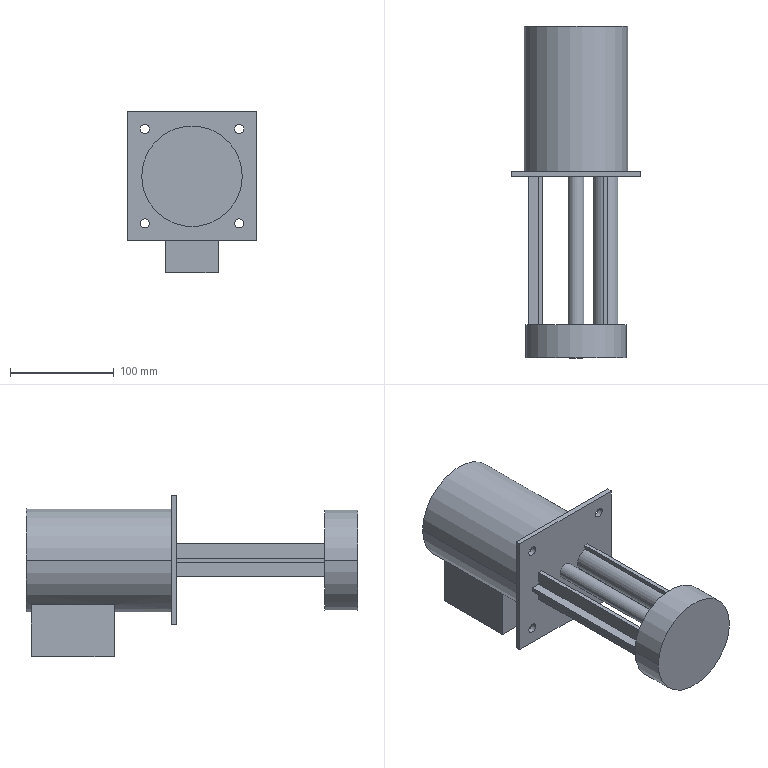Component | SolidWorks | WaterPump-1 | 1 solid | 45 faces | box 125 x 320 x 155.5 mm | volume 1715605 mm3 | plane 28 | cylinder 17 | commonest cylinder face diameters 9 x8 24 x3 100 x2 97 x2 15 x2
build123d program:
from build123d import *

# Parameters (mm, degrees)
SKETCH8_W                = 149
SKETCH8_H                = 149
BOSS_EXTRUDE2_DEPTH      = 5
SKETCH9_R                = 4.5
CUT_EXTRUDE2_DEPTH       = 5
BOSS_EXTRUDE3_DEPTH      = 175
SKETCH11_R               = 7.5
BOSS_EXTRUDE4_DEPTH      = 153
SKETCH12_R               = 48.5
BOSS_EXTRUDE5_DEPTH      = 32
SKETCH13_R               = 50
BOSS_EXTRUDE6_DEPTH      = 140
SKETCH15_W               = 51
SKETCH15_H               = 80
BOSS_EXTRUDE7_DEPTH      = 43
BOSS_EXTRUDE8_REACH      = 334.451
BOSS_EXTRUDE8_END_RADIUS = 50
SKETCH16_W               = 51
SKETCH16_H               = 80
SKETCH17_OUTSIDE_W       = 229.142
SKETCH17_OUTSIDE_H       = 247.642
SKETCH17_OUTSIDE_W_2     = 125
SKETCH17_OUTSIDE_H_2     = 125
CUT_EXTRUDE3_DEPTH       = 10


with BuildPart() as part:
    # Sketch8 → Boss-Extrude2 (new body)
    with BuildSketch(Plane.XY):
        with Locations((-149.258, 88.664)):
            Rectangle(SKETCH8_W, SKETCH8_H)
    extrude(amount=BOSS_EXTRUDE2_DEPTH)

    # Sketch9 → Cut-Extrude2 (cut)
    with BuildSketch(Plane.XY.offset(5)):
        with Locations((-194.758, 134.164)):
            Circle(SKETCH9_R)
        with Locations((-103.758, 134.164)):
            Circle(SKETCH9_R)
        with Locations((-103.758, 43.164)):
            Circle(SKETCH9_R)
        with Locations((-194.758, 43.164)):
            Circle(SKETCH9_R)
    extrude(amount=-CUT_EXTRUDE2_DEPTH, mode=Mode.SUBTRACT)

    # Sketch10 → Boss-Extrude3 (add)
    with BuildSketch(Plane.XY.offset(5)):
        Polygon((-185.758, 104.664), (-181.758, 104.664), (-181.758, 72.664), (-185.758, 72.664), (-185.758, 86.664), (-194.758, 86.664), (-194.758, 90.664), (-185.758, 90.664), align=None)
        with BuildLine():
            Line((-122.758, 104.664), (-118.758, 104.664))
            Line((-118.758, 104.664), (-118.758, 100.496))
            ThreePointArc((-118.758, 100.496), (-108.758, 88.664), (-118.758, 76.832))
            Line((-118.758, 76.832), (-118.758, 72.664))
            Line((-118.758, 72.664), (-122.758, 72.664))
            Line((-122.758, 72.664), (-122.758, 76.832))
            ThreePointArc((-122.758, 76.832), (-132.758, 88.664), (-122.758, 100.496))
            Line((-122.758, 100.496), (-122.758, 104.664))
        make_face()
    extrude(amount=BOSS_EXTRUDE3_DEPTH)

    # Sketch11 → Boss-Extrude4 (add)
    with BuildSketch(Plane.XY.offset(5)):
        with Locations((-149.258, 88.664)):
            Circle(SKETCH11_R)
    extrude(amount=BOSS_EXTRUDE4_DEPTH)

    # Sketch12 → Boss-Extrude5 (add)
    with BuildSketch(Plane.XY.offset(180)):
        with Locations((-149.258, 88.664)):
            Circle(SKETCH12_R)
    extrude(amount=-BOSS_EXTRUDE5_DEPTH)

    # Sketch13 → Boss-Extrude6 (add)
    with BuildSketch(Plane(origin=(0, 0, 0), x_dir=(-1, 0, 0), z_dir=(0, 0, -1))):
        with Locations(Location((149.258, 88.664, 0), (0, 0, 180))):
            Circle(SKETCH13_R)
    extrude(amount=BOSS_EXTRUDE6_DEPTH)



with BuildPart() as body_2:
    # Sketch15 → Boss-Extrude7 (new body)
    with BuildSketch(Plane(origin=(-149.258, 38.664, -140), x_dir=(-1, 0, 0), z_dir=(0, -1, 0))):
        with Locations((0.2199, -45)):
            Rectangle(SKETCH15_W, SKETCH15_H)
    extrude(amount=BOSS_EXTRUDE7_DEPTH)


with BuildPart() as part_1:
    add(part.part)

    add(body_2.part)  # Boss-Extrude8 merges body 2
    # Boss-Extrude8: up to this cylinder (the profile starts outside it)
    boss_extrude8_end = Plane(origin=(-149.258, 88.664, -95), z_dir=(0, 0, 1)) * Cylinder(BOSS_EXTRUDE8_END_RADIUS, 769.902, mode=Mode.PRIVATE)
    # Sketch16 → Boss-Extrude8 (add, up to the surface)
    with BuildSketch(Plane(origin=(0, -4.336, 0), x_dir=(-1, 0, 0), z_dir=(0, -1, 0)), mode=Mode.PRIVATE) as boss_extrude8_sk1:
        with Locations((149.478, 95)):
            Rectangle(SKETCH16_W, SKETCH16_H)
    boss_extrude8_tool1 = extrude(boss_extrude8_sk1.sketch, amount=-BOSS_EXTRUDE8_REACH, mode=Mode.PRIVATE) - boss_extrude8_end
    add(boss_extrude8_tool1.solids().sort_by_distance((-149.478, -4.336, -95))[0])

    # Sketch17 outside → Cut-Extrude3 (cut)
    with BuildSketch(Plane(origin=(0, 0, 0), x_dir=(-1, 0, 0), z_dir=(0, 0, -1))):
        with Locations((149.258, 79.414)):
            Rectangle(SKETCH17_OUTSIDE_W, SKETCH17_OUTSIDE_H)
        with Locations((149.258, 88.664)):
            Rectangle(SKETCH17_OUTSIDE_W_2, SKETCH17_OUTSIDE_H_2, mode=Mode.SUBTRACT)
    extrude(amount=-CUT_EXTRUDE3_DEPTH, mode=Mode.SUBTRACT)


solid = part_1.part

# Placed as in the assembly
solid = solid.moved(Location((820.708, -691.434, -162.183), (90, 0, 0)))